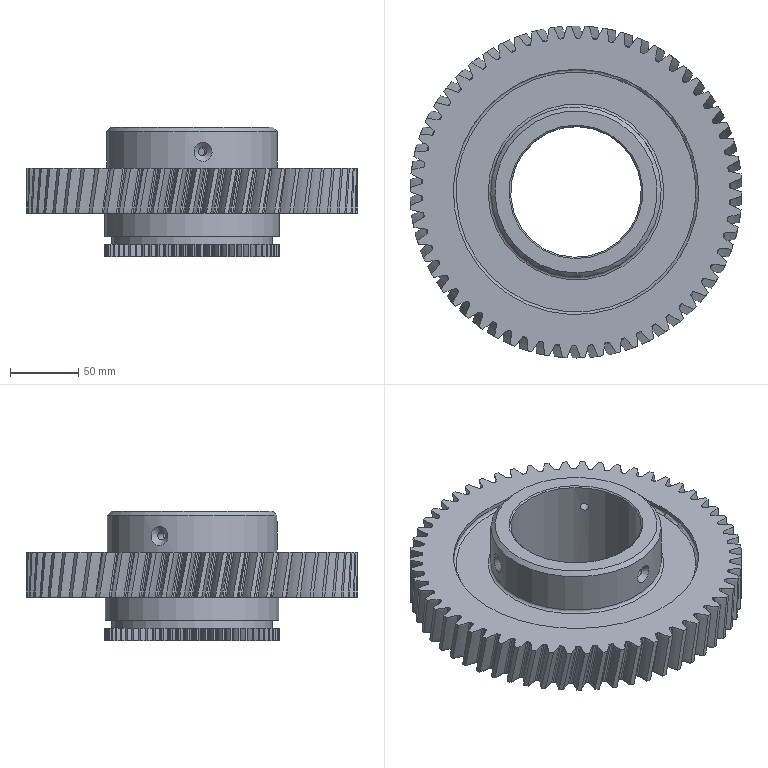Component | NX | CA6140-ZHUZHOU-CHILUN3 | 1 solid | 746 faces | volume 1373907 mm3 | other 310 | spline 290 | cylinder 129 | plane 8 | cone 5 | torus 4 | commonest cylinder face diameters 119 x62 225.579 x58 6 x3 180 x2 96 x1 128 x1 125 x1 118 x1